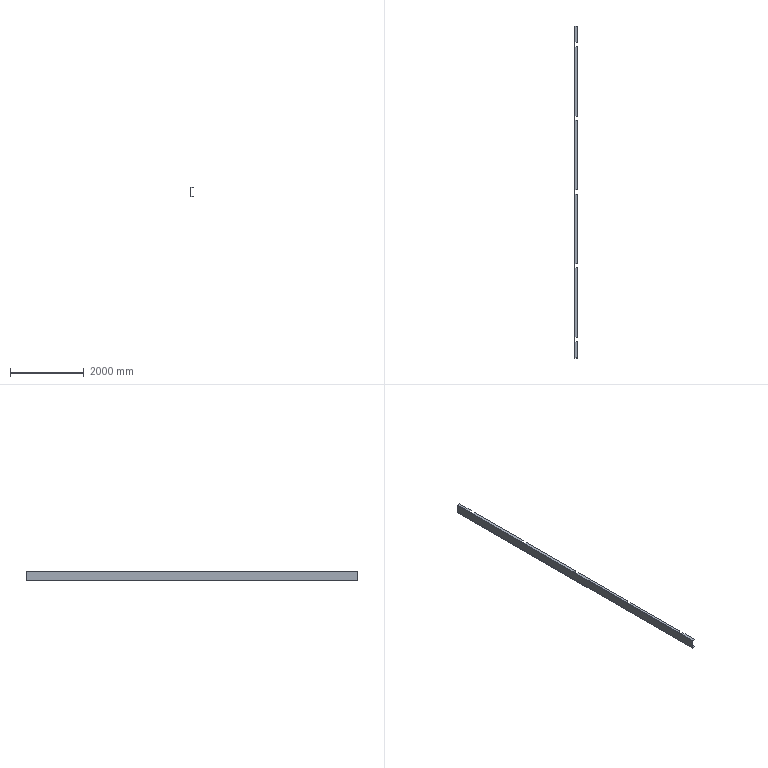Component | NX | CHUNSHUIJINCAO_5_2_2 | 1 solid | 50 faces | volume 34580640 mm3 | plane 50